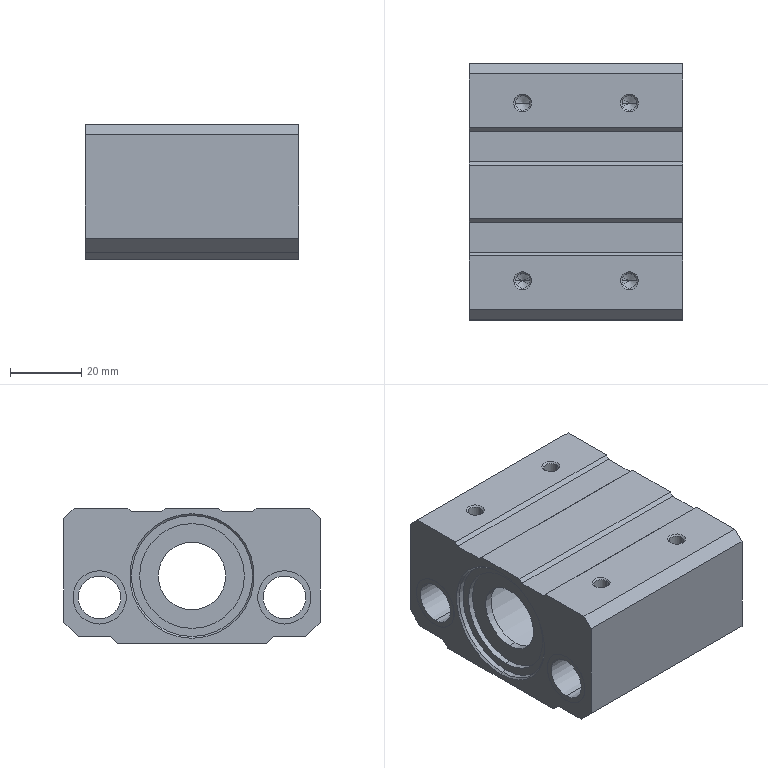Component | SolidWorks | BearingLiftingModule-1_RMT16X100S_0_+_CS1-G-2-1_RMT-16X100-S(0)_body-1 | 1 solid | 106 faces | volume 96471 mm3 | cylinder 42 | plane 36 | cone 28 | commonest cylinder face diameters 15 x8 4.134 x8 29.5 x4 19 x4 34 x4 12 x4 4.6 x4 4 x4